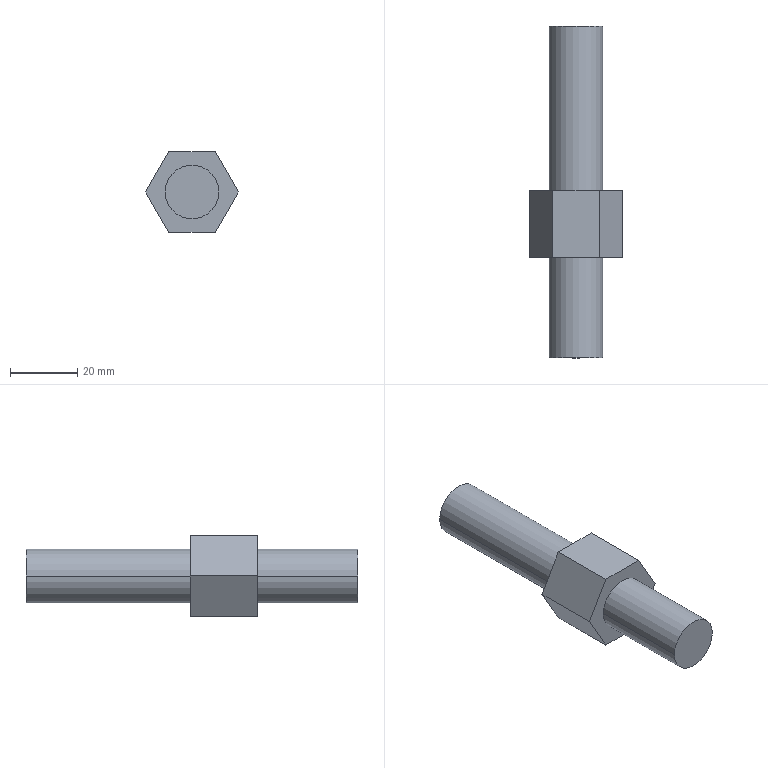Component | SolidWorks | M16LocatingScrew-1 | 1 solid | 14 faces | box 27.71 x 99 x 24 mm | volume 25861 mm3 | plane 10 | cylinder 4 | commonest cylinder face diameters 16 x4
build123d program:
from build123d import *

# Parameters (mm, degrees)
BOSS_EXTRUDE1_DEPTH = 20
SKETCH2_R           = 8
BOSS_EXTRUDE2_DEPTH = 30
BOSS_EXTRUDE3_START = 49
SKETCH3_R           = 8
BOSS_EXTRUDE3_DEPTH = 49


with BuildPart() as part:
    # Sketch1 → Boss-Extrude1 (new body)
    with BuildSketch(Plane.XY):
        Polygon((6.928, 12), (-6.928, 12), (-13.856, 0), (-6.928, -12), (6.928, -12), (13.856, 0), align=None)
    extrude(amount=BOSS_EXTRUDE1_DEPTH)

    # Sketch2 → Boss-Extrude2 (add)
    with BuildSketch(Plane.XY.offset(20)):
        Circle(SKETCH2_R)
    extrude(amount=BOSS_EXTRUDE2_DEPTH)

    # Sketch3 → Boss-Extrude3 (add)
    with BuildSketch(Plane(origin=(0, 0, 0), x_dir=(-1, 0, 0), z_dir=(0, 0, -1)).offset(BOSS_EXTRUDE3_START)):
        with Locations(Location((0, 0, 0), (0, 0, 180))):
            Circle(SKETCH3_R)
    extrude(amount=-BOSS_EXTRUDE3_DEPTH)


solid = part.part

# Placed as in the assembly
solid = solid.moved(Location((30, 956, -40), (90, 0, 0)))
STEP:
#1=COLOUR_RGB('',0.7922,0.8196,0.9333);
#2=FILL_AREA_STYLE_COLOUR('',#1);
#3=FILL_AREA_STYLE('',(#2));
#4=SURFACE_STYLE_FILL_AREA(#3);
#5=SURFACE_SIDE_STYLE('',(#4));
#6=SURFACE_STYLE_USAGE(.BOTH.,#5);
#7=PRESENTATION_STYLE_ASSIGNMENT((#6));
#8=CARTESIAN_POINT('',(0.8661,39.567,-1.575));
#9=VERTEX_POINT('',#8);
#10=CARTESIAN_POINT('',(1.496,39.567,-1.575));
#11=VERTEX_POINT('',#10);
#12=CARTESIAN_POINT('',(1.181,39.567,-1.575));
#13=DIRECTION('',(0.,1.,0.));
#14=DIRECTION('',(-1.,0.,0.));
#15=AXIS2_PLACEMENT_3D('',#12,#13,#14);
#16=CIRCLE('',#15,0.315);
#17=EDGE_CURVE('',#9,#11,#16,.T.);
#18=ORIENTED_EDGE('',*,*,#17,.F.);
#19=CARTESIAN_POINT('',(0.8661,37.638,-1.575));
#20=VERTEX_POINT('',#19);
#21=CARTESIAN_POINT('',(0.8661,39.567,-1.575));
#22=DIRECTION('',(0.,-1.,0.));
#23=VECTOR('',#22,39.37);
#24=LINE('',#21,#23);
#25=EDGE_CURVE('',#9,#20,#24,.T.);
#26=ORIENTED_EDGE('',*,*,#25,.T.);
#27=CARTESIAN_POINT('',(1.496,37.638,-1.575));
#28=VERTEX_POINT('',#27);
#29=CARTESIAN_POINT('',(1.181,37.638,-1.575));
#30=DIRECTION('',(0.,1.,0.));
#31=DIRECTION('',(1.,0.,0.));
#32=AXIS2_PLACEMENT_3D('',#29,#30,#31);
#33=CIRCLE('',#32,0.315);
#34=EDGE_CURVE('',#20,#28,#33,.T.);
#35=ORIENTED_EDGE('',*,*,#34,.T.);
#36=CARTESIAN_POINT('',(1.496,39.567,-1.575));
#37=DIRECTION('',(0.,-1.,0.));
#38=VECTOR('',#37,39.37);
#39=LINE('',#36,#38);
#40=EDGE_CURVE('',#11,#28,#39,.T.);
#41=ORIENTED_EDGE('',*,*,#40,.F.);
#42=EDGE_LOOP('',(#18,#26,#35,#41));
#43=FACE_OUTER_BOUND('',#42,.T.);
#44=CARTESIAN_POINT('',(1.181,39.567,-1.575));
#45=DIRECTION('',(0.,-1.,0.));
#46=DIRECTION('',(1.,0.,0.));
#47=AXIS2_PLACEMENT_3D('',#44,#45,#46);
#48=CYLINDRICAL_SURFACE('',#47,0.315);
#49=ADVANCED_FACE('',(#43),#48,.T.);
#50=CARTESIAN_POINT('',(1.496,35.669,-1.575));
#51=VERTEX_POINT('',#50);
#52=CARTESIAN_POINT('',(0.8661,35.669,-1.575));
#53=VERTEX_POINT('',#52);
#54=CARTESIAN_POINT('',(1.181,35.669,-1.575));
#55=DIRECTION('',(0.,-1.,0.));
#56=DIRECTION('',(1.,0.,0.));
#57=AXIS2_PLACEMENT_3D('',#54,#55,#56);
#58=CIRCLE('',#57,0.315);
#59=EDGE_CURVE('',#51,#53,#58,.T.);
#60=ORIENTED_EDGE('',*,*,#59,.F.);
#61=CARTESIAN_POINT('',(1.496,36.85,-1.575));
#62=VERTEX_POINT('',#61);
#63=CARTESIAN_POINT('',(1.496,35.669,-1.575));
#64=DIRECTION('',(0.,1.,0.));
#65=VECTOR('',#64,39.37);
#66=LINE('',#63,#65);
#67=EDGE_CURVE('',#51,#62,#66,.T.);
#68=ORIENTED_EDGE('',*,*,#67,.T.);
#69=CARTESIAN_POINT('',(0.8661,36.85,-1.575));
#70=VERTEX_POINT('',#69);
#71=CARTESIAN_POINT('',(1.181,36.85,-1.575));
#72=DIRECTION('',(0.,-1.,0.));
#73=DIRECTION('',(1.,0.,0.));
#74=AXIS2_PLACEMENT_3D('',#71,#72,#73);
#75=CIRCLE('',#74,0.315);
#76=EDGE_CURVE('',#62,#70,#75,.T.);
#77=ORIENTED_EDGE('',*,*,#76,.T.);
#78=CARTESIAN_POINT('',(0.8661,35.669,-1.575));
#79=DIRECTION('',(0.,1.,0.));
#80=VECTOR('',#79,39.37);
#81=LINE('',#78,#80);
#82=EDGE_CURVE('',#53,#70,#81,.T.);
#83=ORIENTED_EDGE('',*,*,#82,.F.);
#84=EDGE_LOOP('',(#60,#68,#77,#83));
#85=FACE_OUTER_BOUND('',#84,.T.);
#86=CARTESIAN_POINT('',(1.181,35.669,-1.575));
#87=DIRECTION('',(0.,1.,0.));
#88=DIRECTION('',(-1.,0.,0.));
#89=AXIS2_PLACEMENT_3D('',#86,#87,#88);
#90=CYLINDRICAL_SURFACE('',#89,0.315);
#91=ADVANCED_FACE('',(#85),#90,.T.);
#92=CARTESIAN_POINT('',(1.727,37.638,-1.575));
#93=VERTEX_POINT('',#92);
#94=CARTESIAN_POINT('',(1.454,37.638,-1.102));
#95=VERTEX_POINT('',#94);
#96=CARTESIAN_POINT('',(1.727,37.638,-1.575));
#97=DIRECTION('',(-0.5,0.,0.866));
#98=VECTOR('',#97,39.37);
#99=LINE('',#96,#98);
#100=EDGE_CURVE('',#93,#95,#99,.T.);
#101=ORIENTED_EDGE('',*,*,#100,.F.);
#102=CARTESIAN_POINT('',(1.454,37.638,-2.047));
#103=VERTEX_POINT('',#102);
#104=CARTESIAN_POINT('',(1.454,37.638,-2.047));
#105=DIRECTION('',(0.5,0.,0.866));
#106=VECTOR('',#105,39.37);
#107=LINE('',#104,#106);
#108=EDGE_CURVE('',#103,#93,#107,.T.);
#109=ORIENTED_EDGE('',*,*,#108,.F.);
#110=CARTESIAN_POINT('',(0.9083,37.638,-2.047));
#111=VERTEX_POINT('',#110);
#112=CARTESIAN_POINT('',(0.9083,37.638,-2.047));
#113=DIRECTION('',(1.,0.,-0.));
#114=VECTOR('',#113,39.37);
#115=LINE('',#112,#114);
#116=EDGE_CURVE('',#111,#103,#115,.T.);
#117=ORIENTED_EDGE('',*,*,#116,.F.);
#118=CARTESIAN_POINT('',(0.6356,37.638,-1.575));
#119=VERTEX_POINT('',#118);
#120=CARTESIAN_POINT('',(0.6356,37.638,-1.575));
#121=DIRECTION('',(0.5,0.,-0.866));
#122=VECTOR('',#121,39.37);
#123=LINE('',#120,#122);
#124=EDGE_CURVE('',#119,#111,#123,.T.);
#125=ORIENTED_EDGE('',*,*,#124,.F.);
#126=CARTESIAN_POINT('',(0.9083,37.638,-1.102));
#127=VERTEX_POINT('',#126);
#128=CARTESIAN_POINT('',(0.9083,37.638,-1.102));
#129=DIRECTION('',(-0.5,0.,-0.866));
#130=VECTOR('',#129,39.37);
#131=LINE('',#128,#130);
#132=EDGE_CURVE('',#127,#119,#131,.T.);
#133=ORIENTED_EDGE('',*,*,#132,.F.);
#134=CARTESIAN_POINT('',(1.454,37.638,-1.102));
#135=DIRECTION('',(-1.,0.,0.));
#136=VECTOR('',#135,39.37);
#137=LINE('',#134,#136);
#138=EDGE_CURVE('',#95,#127,#137,.T.);
#139=ORIENTED_EDGE('',*,*,#138,.F.);
#140=EDGE_LOOP('',(#101,#109,#117,#125,#133,#139));
#141=FACE_OUTER_BOUND('',#140,.T.);
#142=CARTESIAN_POINT('',(1.181,37.638,-1.575));
#143=DIRECTION('',(0.,1.,0.));
#144=DIRECTION('',(1.,0.,0.));
#145=AXIS2_PLACEMENT_3D('',#142,#143,#144);
#146=CIRCLE('',#145,0.315);
#147=EDGE_CURVE('',#28,#20,#146,.T.);
#148=ORIENTED_EDGE('',*,*,#147,.F.);
#149=ORIENTED_EDGE('',*,*,#34,.F.);
#150=EDGE_LOOP('',(#148,#149));
#151=FACE_BOUND('',#150,.T.);
#152=CARTESIAN_POINT('',(1.181,37.638,-1.575));
#153=DIRECTION('',(0.,-1.,0.));
#154=DIRECTION('',(1.,0.,0.));
#155=AXIS2_PLACEMENT_3D('',#152,#153,#154);
#156=PLANE('',#155);
#157=ADVANCED_FACE('',(#141,#151),#156,.F.);
#158=CARTESIAN_POINT('',(1.727,36.85,-1.575));
#159=VERTEX_POINT('',#158);
#160=CARTESIAN_POINT('',(1.454,36.85,-1.102));
#161=VERTEX_POINT('',#160);
#162=CARTESIAN_POINT('',(1.727,36.85,-1.575));
#163=DIRECTION('',(-0.5,0.,0.866));
#164=VECTOR('',#163,39.37);
#165=LINE('',#162,#164);
#166=EDGE_CURVE('',#159,#161,#165,.T.);
#167=ORIENTED_EDGE('',*,*,#166,.T.);
#168=CARTESIAN_POINT('',(0.9083,36.85,-1.102));
#169=VERTEX_POINT('',#168);
#170=CARTESIAN_POINT('',(1.454,36.85,-1.102));
#171=DIRECTION('',(-1.,0.,0.));
#172=VECTOR('',#171,39.37);
#173=LINE('',#170,#172);
#174=EDGE_CURVE('',#161,#169,#173,.T.);
#175=ORIENTED_EDGE('',*,*,#174,.T.);
#176=CARTESIAN_POINT('',(0.6356,36.85,-1.575));
#177=VERTEX_POINT('',#176);
#178=CARTESIAN_POINT('',(0.9083,36.85,-1.102));
#179=DIRECTION('',(-0.5,0.,-0.866));
#180=VECTOR('',#179,39.37);
#181=LINE('',#178,#180);
#182=EDGE_CURVE('',#169,#177,#181,.T.);
#183=ORIENTED_EDGE('',*,*,#182,.T.);
#184=CARTESIAN_POINT('',(0.9083,36.85,-2.047));
#185=VERTEX_POINT('',#184);
#186=CARTESIAN_POINT('',(0.6356,36.85,-1.575));
#187=DIRECTION('',(0.5,0.,-0.866));
#188=VECTOR('',#187,39.37);
#189=LINE('',#186,#188);
#190=EDGE_CURVE('',#177,#185,#189,.T.);
#191=ORIENTED_EDGE('',*,*,#190,.T.);
#192=CARTESIAN_POINT('',(1.454,36.85,-2.047));
#193=VERTEX_POINT('',#192);
#194=CARTESIAN_POINT('',(0.9083,36.85,-2.047));
#195=DIRECTION('',(1.,0.,-0.));
#196=VECTOR('',#195,39.37);
#197=LINE('',#194,#196);
#198=EDGE_CURVE('',#185,#193,#197,.T.);
#199=ORIENTED_EDGE('',*,*,#198,.T.);
#200=CARTESIAN_POINT('',(1.454,36.85,-2.047));
#201=DIRECTION('',(0.5,0.,0.866));
#202=VECTOR('',#201,39.37);
#203=LINE('',#200,#202);
#204=EDGE_CURVE('',#193,#159,#203,.T.);
#205=ORIENTED_EDGE('',*,*,#204,.T.);
#206=EDGE_LOOP('',(#167,#175,#183,#191,#199,#205));
#207=FACE_OUTER_BOUND('',#206,.T.);
#208=CARTESIAN_POINT('',(1.181,36.85,-1.575));
#209=DIRECTION('',(0.,-1.,0.));
#210=DIRECTION('',(1.,0.,0.));
#211=AXIS2_PLACEMENT_3D('',#208,#209,#210);
#212=CIRCLE('',#211,0.315);
#213=EDGE_CURVE('',#70,#62,#212,.T.);
#214=ORIENTED_EDGE('',*,*,#213,.F.);
#215=ORIENTED_EDGE('',*,*,#76,.F.);
#216=EDGE_LOOP('',(#214,#215));
#217=FACE_BOUND('',#216,.T.);
#218=CARTESIAN_POINT('',(1.181,36.85,-1.575));
#219=DIRECTION('',(0.,-1.,0.));
#220=DIRECTION('',(1.,0.,0.));
#221=AXIS2_PLACEMENT_3D('',#218,#219,#220);
#222=PLANE('',#221);
#223=ADVANCED_FACE('',(#207,#217),#222,.T.);
#224=ORIENTED_EDGE('',*,*,#100,.T.);
#225=CARTESIAN_POINT('',(1.454,36.85,-1.102));
#226=DIRECTION('',(0.,1.,0.));
#227=VECTOR('',#226,39.37);
#228=LINE('',#225,#227);
#229=EDGE_CURVE('',#161,#95,#228,.T.);
#230=ORIENTED_EDGE('',*,*,#229,.F.);
#231=ORIENTED_EDGE('',*,*,#166,.F.);
#232=CARTESIAN_POINT('',(1.727,36.85,-1.575));
#233=DIRECTION('',(0.,1.,0.));
#234=VECTOR('',#233,39.37);
#235=LINE('',#232,#234);
#236=EDGE_CURVE('',#159,#93,#235,.T.);
#237=ORIENTED_EDGE('',*,*,#236,.T.);
#238=EDGE_LOOP('',(#224,#230,#231,#237));
#239=FACE_OUTER_BOUND('',#238,.T.);
#240=CARTESIAN_POINT('',(1.727,36.85,-1.575));
#241=DIRECTION('',(-0.866,0.,-0.5));
#242=DIRECTION('',(0.5,0.,-0.866));
#243=AXIS2_PLACEMENT_3D('',#240,#241,#242);
#244=PLANE('',#243);
#245=ADVANCED_FACE('',(#239),#244,.F.);
#246=ORIENTED_EDGE('',*,*,#138,.T.);
#247=CARTESIAN_POINT('',(0.9083,36.85,-1.102));
#248=DIRECTION('',(0.,1.,0.));
#249=VECTOR('',#248,39.37);
#250=LINE('',#247,#249);
#251=EDGE_CURVE('',#169,#127,#250,.T.);
#252=ORIENTED_EDGE('',*,*,#251,.F.);
#253=ORIENTED_EDGE('',*,*,#174,.F.);
#254=ORIENTED_EDGE('',*,*,#229,.T.);
#255=EDGE_LOOP('',(#246,#252,#253,#254));
#256=FACE_OUTER_BOUND('',#255,.T.);
#257=CARTESIAN_POINT('',(1.454,36.85,-1.102));
#258=DIRECTION('',(-0.,0.,-1.));
#259=DIRECTION('',(1.,0.,-0.));
#260=AXIS2_PLACEMENT_3D('',#257,#258,#259);
#261=PLANE('',#260);
#262=ADVANCED_FACE('',(#256),#261,.F.);
#263=ORIENTED_EDGE('',*,*,#132,.T.);
#264=CARTESIAN_POINT('',(0.6356,36.85,-1.575));
#265=DIRECTION('',(0.,1.,0.));
#266=VECTOR('',#265,39.37);
#267=LINE('',#264,#266);
#268=EDGE_CURVE('',#177,#119,#267,.T.);
#269=ORIENTED_EDGE('',*,*,#268,.F.);
#270=ORIENTED_EDGE('',*,*,#182,.F.);
#271=ORIENTED_EDGE('',*,*,#251,.T.);
#272=EDGE_LOOP('',(#263,#269,#270,#271));
#273=FACE_OUTER_BOUND('',#272,.T.);
#274=CARTESIAN_POINT('',(0.9083,36.85,-1.102));
#275=DIRECTION('',(0.866,0.,-0.5));
#276=DIRECTION('',(0.5,0.,0.866));
#277=AXIS2_PLACEMENT_3D('',#274,#275,#276);
#278=PLANE('',#277);
#279=ADVANCED_FACE('',(#273),#278,.F.);
#280=ORIENTED_EDGE('',*,*,#124,.T.);
#281=CARTESIAN_POINT('',(0.9083,36.85,-2.047));
#282=DIRECTION('',(0.,1.,0.));
#283=VECTOR('',#282,39.37);
#284=LINE('',#281,#283);
#285=EDGE_CURVE('',#185,#111,#284,.T.);
#286=ORIENTED_EDGE('',*,*,#285,.F.);
#287=ORIENTED_EDGE('',*,*,#190,.F.);
#288=ORIENTED_EDGE('',*,*,#268,.T.);
#289=EDGE_LOOP('',(#280,#286,#287,#288));
#290=FACE_OUTER_BOUND('',#289,.T.);
#291=CARTESIAN_POINT('',(0.6356,36.85,-1.575));
#292=DIRECTION('',(0.866,0.,0.5));
#293=DIRECTION('',(-0.5,0.,0.866));
#294=AXIS2_PLACEMENT_3D('',#291,#292,#293);
#295=PLANE('',#294);
#296=ADVANCED_FACE('',(#290),#295,.F.);
#297=ORIENTED_EDGE('',*,*,#116,.T.);
#298=CARTESIAN_POINT('',(1.454,36.85,-2.047));
#299=DIRECTION('',(0.,1.,0.));
#300=VECTOR('',#299,39.37);
#301=LINE('',#298,#300);
#302=EDGE_CURVE('',#193,#103,#301,.T.);
#303=ORIENTED_EDGE('',*,*,#302,.F.);
#304=ORIENTED_EDGE('',*,*,#198,.F.);
#305=ORIENTED_EDGE('',*,*,#285,.T.);
#306=EDGE_LOOP('',(#297,#303,#304,#305));
#307=FACE_OUTER_BOUND('',#306,.T.);
#308=CARTESIAN_POINT('',(0.9083,36.85,-2.047));
#309=DIRECTION('',(0.,0.,1.));
#310=DIRECTION('',(-1.,0.,0.));
#311=AXIS2_PLACEMENT_3D('',#308,#309,#310);
#312=PLANE('',#311);
#313=ADVANCED_FACE('',(#307),#312,.F.);
#314=ORIENTED_EDGE('',*,*,#108,.T.);
#315=ORIENTED_EDGE('',*,*,#236,.F.);
#316=ORIENTED_EDGE('',*,*,#204,.F.);
#317=ORIENTED_EDGE('',*,*,#302,.T.);
#318=EDGE_LOOP('',(#314,#315,#316,#317));
#319=FACE_OUTER_BOUND('',#318,.T.);
#320=CARTESIAN_POINT('',(1.454,36.85,-2.047));
#321=DIRECTION('',(-0.866,0.,0.5));
#322=DIRECTION('',(-0.5,0.,-0.866));
#323=AXIS2_PLACEMENT_3D('',#320,#321,#322);
#324=PLANE('',#323);
#325=ADVANCED_FACE('',(#319),#324,.F.);
#326=ORIENTED_EDGE('',*,*,#67,.F.);
#327=CARTESIAN_POINT('',(1.181,35.669,-1.575));
#328=DIRECTION('',(0.,-1.,0.));
#329=DIRECTION('',(1.,0.,0.));
#330=AXIS2_PLACEMENT_3D('',#327,#328,#329);
#331=CIRCLE('',#330,0.315);
#332=EDGE_CURVE('',#53,#51,#331,.T.);
#333=ORIENTED_EDGE('',*,*,#332,.F.);
#334=ORIENTED_EDGE('',*,*,#82,.T.);
#335=ORIENTED_EDGE('',*,*,#213,.T.);
#336=EDGE_LOOP('',(#326,#333,#334,#335));
#337=FACE_OUTER_BOUND('',#336,.T.);
#338=CARTESIAN_POINT('',(1.181,35.669,-1.575));
#339=DIRECTION('',(0.,1.,0.));
#340=DIRECTION('',(-1.,0.,0.));
#341=AXIS2_PLACEMENT_3D('',#338,#339,#340);
#342=CYLINDRICAL_SURFACE('',#341,0.315);
#343=ADVANCED_FACE('',(#337),#342,.T.);
#344=ORIENTED_EDGE('',*,*,#332,.T.);
#345=ORIENTED_EDGE('',*,*,#59,.T.);
#346=EDGE_LOOP('',(#344,#345));
#347=FACE_OUTER_BOUND('',#346,.T.);
#348=CARTESIAN_POINT('',(1.181,35.669,-1.575));
#349=DIRECTION('',(0.,-1.,0.));
#350=DIRECTION('',(1.,0.,0.));
#351=AXIS2_PLACEMENT_3D('',#348,#349,#350);
#352=PLANE('',#351);
#353=ADVANCED_FACE('',(#347),#352,.T.);
#354=ORIENTED_EDGE('',*,*,#25,.F.);
#355=CARTESIAN_POINT('',(1.181,39.567,-1.575));
#356=DIRECTION('',(0.,1.,0.));
#357=DIRECTION('',(-1.,0.,0.));
#358=AXIS2_PLACEMENT_3D('',#355,#356,#357);
#359=CIRCLE('',#358,0.315);
#360=EDGE_CURVE('',#11,#9,#359,.T.);
#361=ORIENTED_EDGE('',*,*,#360,.F.);
#362=ORIENTED_EDGE('',*,*,#40,.T.);
#363=ORIENTED_EDGE('',*,*,#147,.T.);
#364=EDGE_LOOP('',(#354,#361,#362,#363));
#365=FACE_OUTER_BOUND('',#364,.T.);
#366=CARTESIAN_POINT('',(1.181,39.567,-1.575));
#367=DIRECTION('',(0.,-1.,0.));
#368=DIRECTION('',(1.,0.,0.));
#369=AXIS2_PLACEMENT_3D('',#366,#367,#368);
#370=CYLINDRICAL_SURFACE('',#369,0.315);
#371=ADVANCED_FACE('',(#365),#370,.T.);
#372=ORIENTED_EDGE('',*,*,#360,.T.);
#373=ORIENTED_EDGE('',*,*,#17,.T.);
#374=EDGE_LOOP('',(#372,#373));
#375=FACE_OUTER_BOUND('',#374,.T.);
#376=CARTESIAN_POINT('',(1.181,39.567,-1.575));
#377=DIRECTION('',(0.,1.,0.));
#378=DIRECTION('',(-1.,0.,0.));
#379=AXIS2_PLACEMENT_3D('',#376,#377,#378);
#380=PLANE('',#379);
#381=ADVANCED_FACE('',(#375),#380,.T.);
#382=CLOSED_SHELL('',(#49,#91,#157,#223,#245,#262,#279,#296,#313,#325,#343,#353,#371,#381));
#383=MANIFOLD_SOLID_BREP('',#382);
#384=STYLED_ITEM('',(#7),#383);
#385=PRESENTATION_LAYER_ASSIGNMENT('','',(#384));
#386=(LENGTH_UNIT()NAMED_UNIT(*)SI_UNIT($,.METRE.));
#387=LENGTH_MEASURE_WITH_UNIT(LENGTH_MEASURE(0.0254),#386);
#388=DIMENSIONAL_EXPONENTS(1.,0.,0.,0.,0.,0.,0.);
#389=(CONVERSION_BASED_UNIT('',#387)LENGTH_UNIT()NAMED_UNIT(#388));
#390=UNCERTAINTY_MEASURE_WITH_UNIT(LENGTH_MEASURE(0.00001),#389,'','');
#391=(NAMED_UNIT(*)PLANE_ANGLE_UNIT()SI_UNIT($,.RADIAN.));
#392=(NAMED_UNIT(*)SI_UNIT($,.STERADIAN.)SOLID_ANGLE_UNIT());
#393=(GEOMETRIC_REPRESENTATION_CONTEXT(3)GLOBAL_UNCERTAINTY_ASSIGNED_CONTEXT((#390))GLOBAL_UNIT_ASSIGNED_CONTEXT((#389,#391,#392))REPRESENTATION_CONTEXT('',''));
#394=MECHANICAL_DESIGN_GEOMETRIC_PRESENTATION_REPRESENTATION('',(#384),#393);
#395=CARTESIAN_POINT('',(0.,0.,0.));
#396=DIRECTION('',(0.,0.,1.));
#397=DIRECTION('',(1.,0.,0.));
#398=AXIS2_PLACEMENT_3D('',#395,#396,#397);
#399=(LENGTH_UNIT()NAMED_UNIT(*)SI_UNIT($,.METRE.));
#400=LENGTH_MEASURE_WITH_UNIT(LENGTH_MEASURE(0.0254),#399);
#401=DIMENSIONAL_EXPONENTS(1.,0.,0.,0.,0.,0.,0.);
#402=(CONVERSION_BASED_UNIT('',#400)LENGTH_UNIT()NAMED_UNIT(#401));
#403=UNCERTAINTY_MEASURE_WITH_UNIT(LENGTH_MEASURE(0.00001),#402,'','');
#404=(NAMED_UNIT(*)PLANE_ANGLE_UNIT()SI_UNIT($,.RADIAN.));
#405=(NAMED_UNIT(*)SI_UNIT($,.STERADIAN.)SOLID_ANGLE_UNIT());
#406=(GEOMETRIC_REPRESENTATION_CONTEXT(3)GLOBAL_UNCERTAINTY_ASSIGNED_CONTEXT((#403))GLOBAL_UNIT_ASSIGNED_CONTEXT((#402,#404,#405))REPRESENTATION_CONTEXT('',''));
#407=ADVANCED_BREP_SHAPE_REPRESENTATION('',(#383,#398),#406);